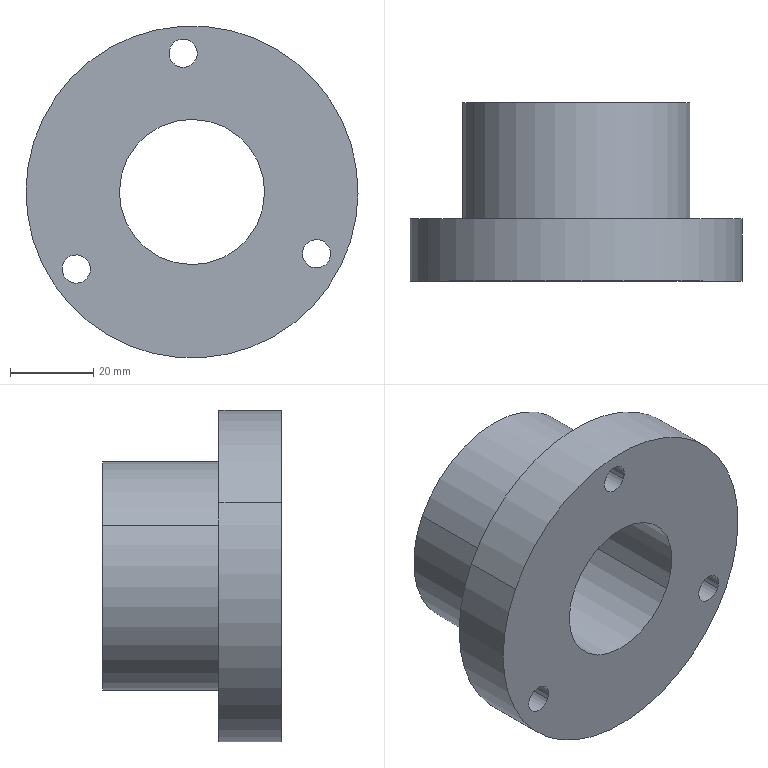Component | SolidWorks | BearingHousing2-1 | 1 solid | 18 faces | box 80 x 43 x 80 mm | volume 88097 mm3 | cylinder 14 | plane 4 | commonest cylinder face diameters 6.8 x6 80 x2 35 x2 47 x2 55 x2
STEP:
#1=COLOUR_RGB('',0.7922,0.8196,0.9333);
#2=FILL_AREA_STYLE_COLOUR('',#1);
#3=FILL_AREA_STYLE('',(#2));
#4=SURFACE_STYLE_FILL_AREA(#3);
#5=SURFACE_SIDE_STYLE('',(#4));
#6=SURFACE_STYLE_USAGE(.BOTH.,#5);
#7=PRESENTATION_STYLE_ASSIGNMENT((#6));
#8=CARTESIAN_POINT('',(-7.394,18.149,5.891));
#9=VERTEX_POINT('',#8);
#10=CARTESIAN_POINT('',(-7.154,18.149,5.772));
#11=VERTEX_POINT('',#10);
#12=CARTESIAN_POINT('',(-7.274,18.149,5.832));
#13=DIRECTION('',(0.,1.,0.));
#14=DIRECTION('',(0.896,0.,-0.4441));
#15=AXIS2_PLACEMENT_3D('',#12,#13,#14);
#16=CIRCLE('',#15,0.1339);
#17=EDGE_CURVE('',#9,#11,#16,.T.);
#18=ORIENTED_EDGE('',*,*,#17,.T.);
#19=CARTESIAN_POINT('',(-7.154,17.558,5.772));
#20=VERTEX_POINT('',#19);
#21=CARTESIAN_POINT('',(-7.154,17.558,5.772));
#22=DIRECTION('',(0.,-1.,0.));
#23=VECTOR('',#22,39.37);
#24=LINE('',#21,#23);
#25=EDGE_CURVE('',#11,#20,#24,.T.);
#26=ORIENTED_EDGE('',*,*,#25,.T.);
#27=CARTESIAN_POINT('',(-7.394,17.558,5.891));
#28=VERTEX_POINT('',#27);
#29=CARTESIAN_POINT('',(-7.274,17.558,5.832));
#30=DIRECTION('',(0.,-1.,0.));
#31=DIRECTION('',(-0.896,0.,0.4441));
#32=AXIS2_PLACEMENT_3D('',#29,#30,#31);
#33=CIRCLE('',#32,0.1339);
#34=EDGE_CURVE('',#20,#28,#33,.T.);
#35=ORIENTED_EDGE('',*,*,#34,.T.);
#36=CARTESIAN_POINT('',(-7.394,17.558,5.891));
#37=DIRECTION('',(0.,-1.,0.));
#38=VECTOR('',#37,39.37);
#39=LINE('',#36,#38);
#40=EDGE_CURVE('',#9,#28,#39,.T.);
#41=ORIENTED_EDGE('',*,*,#40,.F.);
#42=EDGE_LOOP('',(#18,#26,#35,#41));
#43=FACE_OUTER_BOUND('',#42,.T.);
#44=CARTESIAN_POINT('',(-7.274,17.558,5.832));
#45=DIRECTION('',(0.,-1.,0.));
#46=DIRECTION('',(-0.896,0.,0.4441));
#47=AXIS2_PLACEMENT_3D('',#44,#45,#46);
#48=CYLINDRICAL_SURFACE('',#47,0.1339);
#49=ADVANCED_FACE('',(#43),#48,.F.);
#50=CARTESIAN_POINT('',(-8.66,18.149,7.793));
#51=VERTEX_POINT('',#50);
#52=CARTESIAN_POINT('',(-8.42,18.149,7.674));
#53=VERTEX_POINT('',#52);
#54=CARTESIAN_POINT('',(-8.54,18.149,7.734));
#55=DIRECTION('',(0.,1.,0.));
#56=DIRECTION('',(0.896,0.,-0.4441));
#57=AXIS2_PLACEMENT_3D('',#54,#55,#56);
#58=CIRCLE('',#57,0.1339);
#59=EDGE_CURVE('',#51,#53,#58,.T.);
#60=ORIENTED_EDGE('',*,*,#59,.T.);
#61=CARTESIAN_POINT('',(-8.42,17.558,7.674));
#62=VERTEX_POINT('',#61);
#63=CARTESIAN_POINT('',(-8.42,17.558,7.674));
#64=DIRECTION('',(0.,-1.,0.));
#65=VECTOR('',#64,39.37);
#66=LINE('',#63,#65);
#67=EDGE_CURVE('',#53,#62,#66,.T.);
#68=ORIENTED_EDGE('',*,*,#67,.T.);
#69=CARTESIAN_POINT('',(-8.66,17.558,7.793));
#70=VERTEX_POINT('',#69);
#71=CARTESIAN_POINT('',(-8.54,17.558,7.734));
#72=DIRECTION('',(0.,-1.,0.));
#73=DIRECTION('',(-0.896,0.,0.4441));
#74=AXIS2_PLACEMENT_3D('',#71,#72,#73);
#75=CIRCLE('',#74,0.1339);
#76=EDGE_CURVE('',#62,#70,#75,.T.);
#77=ORIENTED_EDGE('',*,*,#76,.T.);
#78=CARTESIAN_POINT('',(-8.66,17.558,7.793));
#79=DIRECTION('',(0.,-1.,0.));
#80=VECTOR('',#79,39.37);
#81=LINE('',#78,#80);
#82=EDGE_CURVE('',#51,#70,#81,.T.);
#83=ORIENTED_EDGE('',*,*,#82,.F.);
#84=EDGE_LOOP('',(#60,#68,#77,#83));
#85=FACE_OUTER_BOUND('',#84,.T.);
#86=CARTESIAN_POINT('',(-8.54,17.558,7.734));
#87=DIRECTION('',(0.,-1.,0.));
#88=DIRECTION('',(-0.896,0.,0.4441));
#89=AXIS2_PLACEMENT_3D('',#86,#87,#88);
#90=CYLINDRICAL_SURFACE('',#89,0.1339);
#91=ADVANCED_FACE('',(#85),#90,.F.);
#92=CARTESIAN_POINT('',(-9.674,18.149,5.746));
#93=VERTEX_POINT('',#92);
#94=CARTESIAN_POINT('',(-9.434,18.149,5.627));
#95=VERTEX_POINT('',#94);
#96=CARTESIAN_POINT('',(-9.554,18.149,5.687));
#97=DIRECTION('',(0.,1.,0.));
#98=DIRECTION('',(0.896,0.,-0.4441));
#99=AXIS2_PLACEMENT_3D('',#96,#97,#98);
#100=CIRCLE('',#99,0.1339);
#101=EDGE_CURVE('',#93,#95,#100,.T.);
#102=ORIENTED_EDGE('',*,*,#101,.T.);
#103=CARTESIAN_POINT('',(-9.434,17.558,5.627));
#104=VERTEX_POINT('',#103);
#105=CARTESIAN_POINT('',(-9.434,17.558,5.627));
#106=DIRECTION('',(0.,-1.,0.));
#107=VECTOR('',#106,39.37);
#108=LINE('',#105,#107);
#109=EDGE_CURVE('',#95,#104,#108,.T.);
#110=ORIENTED_EDGE('',*,*,#109,.T.);
#111=CARTESIAN_POINT('',(-9.674,17.558,5.746));
#112=VERTEX_POINT('',#111);
#113=CARTESIAN_POINT('',(-9.554,17.558,5.687));
#114=DIRECTION('',(0.,-1.,0.));
#115=DIRECTION('',(-0.896,0.,0.4441));
#116=AXIS2_PLACEMENT_3D('',#113,#114,#115);
#117=CIRCLE('',#116,0.1339);
#118=EDGE_CURVE('',#104,#112,#117,.T.);
#119=ORIENTED_EDGE('',*,*,#118,.T.);
#120=CARTESIAN_POINT('',(-9.674,17.558,5.746));
#121=DIRECTION('',(0.,-1.,0.));
#122=VECTOR('',#121,39.37);
#123=LINE('',#120,#122);
#124=EDGE_CURVE('',#93,#112,#123,.T.);
#125=ORIENTED_EDGE('',*,*,#124,.F.);
#126=EDGE_LOOP('',(#102,#110,#119,#125));
#127=FACE_OUTER_BOUND('',#126,.T.);
#128=CARTESIAN_POINT('',(-9.554,17.558,5.687));
#129=DIRECTION('',(0.,-1.,0.));
#130=DIRECTION('',(-0.896,0.,0.4441));
#131=AXIS2_PLACEMENT_3D('',#128,#129,#130);
#132=CYLINDRICAL_SURFACE('',#131,0.1339);
#133=ADVANCED_FACE('',(#127),#132,.F.);
#134=CARTESIAN_POINT('',(-9.867,18.149,7.117));
#135=VERTEX_POINT('',#134);
#136=CARTESIAN_POINT('',(-7.045,18.149,5.718));
#137=VERTEX_POINT('',#136);
#138=CARTESIAN_POINT('',(-8.456,18.149,6.417));
#139=DIRECTION('',(0.,-1.,0.));
#140=DIRECTION('',(-0.896,0.,0.4441));
#141=AXIS2_PLACEMENT_3D('',#138,#139,#140);
#142=CIRCLE('',#141,1.575);
#143=EDGE_CURVE('',#135,#137,#142,.T.);
#144=ORIENTED_EDGE('',*,*,#143,.T.);
#145=CARTESIAN_POINT('',(-7.045,17.558,5.718));
#146=VERTEX_POINT('',#145);
#147=CARTESIAN_POINT('',(-7.045,17.335,5.718));
#148=DIRECTION('',(0.,-1.,0.));
#149=VECTOR('',#148,39.37);
#150=LINE('',#147,#149);
#151=EDGE_CURVE('',#137,#146,#150,.T.);
#152=ORIENTED_EDGE('',*,*,#151,.T.);
#153=CARTESIAN_POINT('',(-9.867,17.558,7.117));
#154=VERTEX_POINT('',#153);
#155=CARTESIAN_POINT('',(-8.456,17.558,6.417));
#156=DIRECTION('',(0.,-1.,0.));
#157=DIRECTION('',(-0.896,0.,0.4441));
#158=AXIS2_PLACEMENT_3D('',#155,#156,#157);
#159=CIRCLE('',#158,1.575);
#160=EDGE_CURVE('',#154,#146,#159,.T.);
#161=ORIENTED_EDGE('',*,*,#160,.F.);
#162=CARTESIAN_POINT('',(-9.867,17.335,7.117));
#163=DIRECTION('',(0.,-1.,0.));
#164=VECTOR('',#163,39.37);
#165=LINE('',#162,#164);
#166=EDGE_CURVE('',#135,#154,#165,.T.);
#167=ORIENTED_EDGE('',*,*,#166,.F.);
#168=EDGE_LOOP('',(#144,#152,#161,#167));
#169=FACE_OUTER_BOUND('',#168,.T.);
#170=CARTESIAN_POINT('',(-8.456,17.335,6.417));
#171=DIRECTION('',(0.,-1.,0.));
#172=DIRECTION('',(-0.896,0.,0.4441));
#173=AXIS2_PLACEMENT_3D('',#170,#171,#172);
#174=CYLINDRICAL_SURFACE('',#173,1.575);
#175=ADVANCED_FACE('',(#169),#174,.T.);
#176=CARTESIAN_POINT('',(-7.839,18.7,6.111));
#177=VERTEX_POINT('',#176);
#178=CARTESIAN_POINT('',(-9.073,18.7,6.723));
#179=VERTEX_POINT('',#178);
#180=CARTESIAN_POINT('',(-8.456,18.7,6.417));
#181=DIRECTION('',(0.,-1.,0.));
#182=DIRECTION('',(-0.896,0.,0.4441));
#183=AXIS2_PLACEMENT_3D('',#180,#181,#182);
#184=CIRCLE('',#183,0.689);
#185=EDGE_CURVE('',#177,#179,#184,.T.);
#186=ORIENTED_EDGE('',*,*,#185,.F.);
#187=CARTESIAN_POINT('',(-7.839,17.558,6.111));
#188=VERTEX_POINT('',#187);
#189=CARTESIAN_POINT('',(-7.839,17.335,6.111));
#190=DIRECTION('',(0.,-1.,0.));
#191=VECTOR('',#190,39.37);
#192=LINE('',#189,#191);
#193=EDGE_CURVE('',#177,#188,#192,.T.);
#194=ORIENTED_EDGE('',*,*,#193,.T.);
#195=CARTESIAN_POINT('',(-9.073,17.558,6.723));
#196=VERTEX_POINT('',#195);
#197=CARTESIAN_POINT('',(-8.456,17.558,6.417));
#198=DIRECTION('',(0.,-1.,0.));
#199=DIRECTION('',(-0.896,0.,0.4441));
#200=AXIS2_PLACEMENT_3D('',#197,#198,#199);
#201=CIRCLE('',#200,0.689);
#202=EDGE_CURVE('',#188,#196,#201,.T.);
#203=ORIENTED_EDGE('',*,*,#202,.T.);
#204=CARTESIAN_POINT('',(-9.073,17.335,6.723));
#205=DIRECTION('',(0.,-1.,0.));
#206=VECTOR('',#205,39.37);
#207=LINE('',#204,#206);
#208=EDGE_CURVE('',#179,#196,#207,.T.);
#209=ORIENTED_EDGE('',*,*,#208,.F.);
#210=EDGE_LOOP('',(#186,#194,#203,#209));
#211=FACE_OUTER_BOUND('',#210,.T.);
#212=CARTESIAN_POINT('',(-8.456,17.335,6.417));
#213=DIRECTION('',(0.,-1.,0.));
#214=DIRECTION('',(-0.896,0.,0.4441));
#215=AXIS2_PLACEMENT_3D('',#212,#213,#214);
#216=CYLINDRICAL_SURFACE('',#215,0.689);
#217=ADVANCED_FACE('',(#211),#216,.F.);
#218=CARTESIAN_POINT('',(-7.627,19.251,6.006));
#219=VERTEX_POINT('',#218);
#220=CARTESIAN_POINT('',(-9.285,19.251,6.828));
#221=VERTEX_POINT('',#220);
#222=CARTESIAN_POINT('',(-8.456,19.251,6.417));
#223=DIRECTION('',(0.,-1.,0.));
#224=DIRECTION('',(-0.896,0.,0.4441));
#225=AXIS2_PLACEMENT_3D('',#222,#223,#224);
#226=CIRCLE('',#225,0.9252);
#227=EDGE_CURVE('',#219,#221,#226,.T.);
#228=ORIENTED_EDGE('',*,*,#227,.F.);
#229=CARTESIAN_POINT('',(-7.627,18.7,6.006));
#230=VERTEX_POINT('',#229);
#231=CARTESIAN_POINT('',(-7.627,17.335,6.006));
#232=DIRECTION('',(0.,-1.,0.));
#233=VECTOR('',#232,39.37);
#234=LINE('',#231,#233);
#235=EDGE_CURVE('',#219,#230,#234,.T.);
#236=ORIENTED_EDGE('',*,*,#235,.T.);
#237=CARTESIAN_POINT('',(-9.285,18.7,6.828));
#238=VERTEX_POINT('',#237);
#239=CARTESIAN_POINT('',(-8.456,18.7,6.417));
#240=DIRECTION('',(0.,-1.,0.));
#241=DIRECTION('',(-0.896,0.,0.4441));
#242=AXIS2_PLACEMENT_3D('',#239,#240,#241);
#243=CIRCLE('',#242,0.9252);
#244=EDGE_CURVE('',#230,#238,#243,.T.);
#245=ORIENTED_EDGE('',*,*,#244,.T.);
#246=CARTESIAN_POINT('',(-9.285,17.335,6.828));
#247=DIRECTION('',(0.,-1.,0.));
#248=VECTOR('',#247,39.37);
#249=LINE('',#246,#248);
#250=EDGE_CURVE('',#221,#238,#249,.T.);
#251=ORIENTED_EDGE('',*,*,#250,.F.);
#252=EDGE_LOOP('',(#228,#236,#245,#251));
#253=FACE_OUTER_BOUND('',#252,.T.);
#254=CARTESIAN_POINT('',(-8.456,17.335,6.417));
#255=DIRECTION('',(0.,-1.,0.));
#256=DIRECTION('',(-0.896,0.,0.4441));
#257=AXIS2_PLACEMENT_3D('',#254,#255,#256);
#258=CYLINDRICAL_SURFACE('',#257,0.9252);
#259=ADVANCED_FACE('',(#253),#258,.F.);
#260=CARTESIAN_POINT('',(-9.426,19.251,6.898));
#261=VERTEX_POINT('',#260);
#262=CARTESIAN_POINT('',(-7.486,19.251,5.937));
#263=VERTEX_POINT('',#262);
#264=CARTESIAN_POINT('',(-8.456,19.251,6.417));
#265=DIRECTION('',(0.,-1.,0.));
#266=DIRECTION('',(-0.896,0.,0.4441));
#267=AXIS2_PLACEMENT_3D('',#264,#265,#266);
#268=CIRCLE('',#267,1.083);
#269=EDGE_CURVE('',#261,#263,#268,.T.);
#270=ORIENTED_EDGE('',*,*,#269,.T.);
#271=CARTESIAN_POINT('',(-7.486,18.149,5.937));
#272=VERTEX_POINT('',#271);
#273=CARTESIAN_POINT('',(-7.486,17.335,5.937));
#274=DIRECTION('',(0.,-1.,0.));
#275=VECTOR('',#274,39.37);
#276=LINE('',#273,#275);
#277=EDGE_CURVE('',#263,#272,#276,.T.);
#278=ORIENTED_EDGE('',*,*,#277,.T.);
#279=CARTESIAN_POINT('',(-9.426,18.149,6.898));
#280=VERTEX_POINT('',#279);
#281=CARTESIAN_POINT('',(-8.456,18.149,6.417));
#282=DIRECTION('',(0.,-1.,0.));
#283=DIRECTION('',(-0.896,0.,0.4441));
#284=AXIS2_PLACEMENT_3D('',#281,#282,#283);
#285=CIRCLE('',#284,1.083);
#286=EDGE_CURVE('',#280,#272,#285,.T.);
#287=ORIENTED_EDGE('',*,*,#286,.F.);
#288=CARTESIAN_POINT('',(-9.426,17.335,6.898));
#289=DIRECTION('',(0.,-1.,0.));
#290=VECTOR('',#289,39.37);
#291=LINE('',#288,#290);
#292=EDGE_CURVE('',#261,#280,#291,.T.);
#293=ORIENTED_EDGE('',*,*,#292,.F.);
#294=EDGE_LOOP('',(#270,#278,#287,#293));
#295=FACE_OUTER_BOUND('',#294,.T.);
#296=CARTESIAN_POINT('',(-8.456,17.335,6.417));
#297=DIRECTION('',(0.,-1.,0.));
#298=DIRECTION('',(-0.896,0.,0.4441));
#299=AXIS2_PLACEMENT_3D('',#296,#297,#298);
#300=CYLINDRICAL_SURFACE('',#299,1.083);
#301=ADVANCED_FACE('',(#295),#300,.T.);
#302=ORIENTED_EDGE('',*,*,#277,.F.);
#303=CARTESIAN_POINT('',(-8.456,19.251,6.417));
#304=DIRECTION('',(0.,-1.,0.));
#305=DIRECTION('',(-0.896,0.,0.4441));
#306=AXIS2_PLACEMENT_3D('',#303,#304,#305);
#307=CIRCLE('',#306,1.083);
#308=EDGE_CURVE('',#263,#261,#307,.T.);
#309=ORIENTED_EDGE('',*,*,#308,.T.);
#310=ORIENTED_EDGE('',*,*,#292,.T.);
#311=CARTESIAN_POINT('',(-8.456,18.149,6.417));
#312=DIRECTION('',(0.,-1.,0.));
#313=DIRECTION('',(-0.896,0.,0.4441));
#314=AXIS2_PLACEMENT_3D('',#311,#312,#313);
#315=CIRCLE('',#314,1.083);
#316=EDGE_CURVE('',#272,#280,#315,.T.);
#317=ORIENTED_EDGE('',*,*,#316,.F.);
#318=EDGE_LOOP('',(#302,#309,#310,#317));
#319=FACE_OUTER_BOUND('',#318,.T.);
#320=CARTESIAN_POINT('',(-8.456,17.335,6.417));
#321=DIRECTION('',(0.,-1.,0.));
#322=DIRECTION('',(-0.896,0.,0.4441));
#323=AXIS2_PLACEMENT_3D('',#320,#321,#322);
#324=CYLINDRICAL_SURFACE('',#323,1.083);
#325=ADVANCED_FACE('',(#319),#324,.T.);
#326=CARTESIAN_POINT('',(-8.456,19.251,6.417));
#327=DIRECTION('',(0.,-1.,0.));
#328=DIRECTION('',(-0.896,0.,0.4441));
#329=AXIS2_PLACEMENT_3D('',#326,#327,#328);
#330=CIRCLE('',#329,0.9252);
#331=EDGE_CURVE('',#221,#219,#330,.T.);
#332=ORIENTED_EDGE('',*,*,#331,.T.);
#333=ORIENTED_EDGE('',*,*,#227,.T.);
#334=EDGE_LOOP('',(#332,#333));
#335=FACE_BOUND('',#334,.T.);
#336=ORIENTED_EDGE('',*,*,#269,.F.);
#337=ORIENTED_EDGE('',*,*,#308,.F.);
#338=EDGE_LOOP('',(#336,#337));
#339=FACE_OUTER_BOUND('',#338,.T.);
#340=CARTESIAN_POINT('',(-9.285,19.251,6.828));
#341=DIRECTION('',(0.,1.,0.));
#342=DIRECTION('',(0.896,0.,-0.4441));
#343=AXIS2_PLACEMENT_3D('',#340,#341,#342);
#344=PLANE('',#343);
#345=ADVANCED_FACE('',(#335,#339),#344,.T.);
#346=ORIENTED_EDGE('',*,*,#235,.F.);
#347=ORIENTED_EDGE('',*,*,#331,.F.);
#348=ORIENTED_EDGE('',*,*,#250,.T.);
#349=CARTESIAN_POINT('',(-8.456,18.7,6.417));
#350=DIRECTION('',(0.,-1.,0.));
#351=DIRECTION('',(-0.896,0.,0.4441));
#352=AXIS2_PLACEMENT_3D('',#349,#350,#351);
#353=CIRCLE('',#352,0.9252);
#354=EDGE_CURVE('',#238,#230,#353,.T.);
#355=ORIENTED_EDGE('',*,*,#354,.T.);
#356=EDGE_LOOP('',(#346,#347,#348,#355));
#357=FACE_OUTER_BOUND('',#356,.T.);
#358=CARTESIAN_POINT('',(-8.456,17.335,6.417));
#359=DIRECTION('',(0.,-1.,0.));
#360=DIRECTION('',(-0.896,0.,0.4441));
#361=AXIS2_PLACEMENT_3D('',#358,#359,#360);
#362=CYLINDRICAL_SURFACE('',#361,0.9252);
#363=ADVANCED_FACE('',(#357),#362,.F.);
#364=CARTESIAN_POINT('',(-8.456,18.7,6.417));
#365=DIRECTION('',(0.,-1.,0.));
#366=DIRECTION('',(-0.896,0.,0.4441));
#367=AXIS2_PLACEMENT_3D('',#364,#365,#366);
#368=CIRCLE('',#367,0.689);
#369=EDGE_CURVE('',#179,#177,#368,.T.);
#370=ORIENTED_EDGE('',*,*,#369,.T.);
#371=ORIENTED_EDGE('',*,*,#185,.T.);
#372=EDGE_LOOP('',(#370,#371));
#373=FACE_BOUND('',#372,.T.);
#374=ORIENTED_EDGE('',*,*,#354,.F.);
#375=ORIENTED_EDGE('',*,*,#244,.F.);
#376=EDGE_LOOP('',(#374,#375));
#377=FACE_OUTER_BOUND('',#376,.T.);
#378=CARTESIAN_POINT('',(-9.285,18.7,6.828));
#379=DIRECTION('',(0.,1.,0.));
#380=DIRECTION('',(0.896,0.,-0.4441));
#381=AXIS2_PLACEMENT_3D('',#378,#379,#380);
#382=PLANE('',#381);
#383=ADVANCED_FACE('',(#373,#377),#382,.T.);
#384=ORIENTED_EDGE('',*,*,#193,.F.);
#385=ORIENTED_EDGE('',*,*,#369,.F.);
#386=ORIENTED_EDGE('',*,*,#208,.T.);
#387=CARTESIAN_POINT('',(-8.456,17.558,6.417));
#388=DIRECTION('',(0.,-1.,0.));
#389=DIRECTION('',(-0.896,0.,0.4441));
#390=AXIS2_PLACEMENT_3D('',#387,#388,#389);
#391=CIRCLE('',#390,0.689);
#392=EDGE_CURVE('',#196,#188,#391,.T.);
#393=ORIENTED_EDGE('',*,*,#392,.T.);
#394=EDGE_LOOP('',(#384,#385,#386,#393));
#395=FACE_OUTER_BOUND('',#394,.T.);
#396=CARTESIAN_POINT('',(-8.456,17.335,6.417));
#397=DIRECTION('',(0.,-1.,0.));
#398=DIRECTION('',(-0.896,0.,0.4441));
#399=AXIS2_PLACEMENT_3D('',#396,#397,#398);
#400=CYLINDRICAL_SURFACE('',#399,0.689);
#401=ADVANCED_FACE('',(#395),#400,.F.);
#402=CARTESIAN_POINT('',(-7.274,17.558,5.832));
#403=DIRECTION('',(0.,-1.,0.));
#404=DIRECTION('',(-0.896,0.,0.4441));
#405=AXIS2_PLACEMENT_3D('',#402,#403,#404);
#406=CIRCLE('',#405,0.1339);
#407=EDGE_CURVE('',#28,#20,#406,.T.);
#408=ORIENTED_EDGE('',*,*,#407,.F.);
#409=ORIENTED_EDGE('',*,*,#34,.F.);
#410=EDGE_LOOP('',(#408,#409));
#411=FACE_BOUND('',#410,.T.);
#412=CARTESIAN_POINT('',(-8.54,17.558,7.734));
#413=DIRECTION('',(0.,-1.,0.));
#414=DIRECTION('',(-0.896,0.,0.4441));
#415=AXIS2_PLACEMENT_3D('',#412,#413,#414);
#416=CIRCLE('',#415,0.1339);
#417=EDGE_CURVE('',#70,#62,#416,.T.);
#418=ORIENTED_EDGE('',*,*,#417,.F.);
#419=ORIENTED_EDGE('',*,*,#76,.F.);
#420=EDGE_LOOP('',(#418,#419));
#421=FACE_BOUND('',#420,.T.);
#422=CARTESIAN_POINT('',(-9.554,17.558,5.687));
#423=DIRECTION('',(0.,-1.,0.));
#424=DIRECTION('',(-0.896,0.,0.4441));
#425=AXIS2_PLACEMENT_3D('',#422,#423,#424);
#426=CIRCLE('',#425,0.1339);
#427=EDGE_CURVE('',#112,#104,#426,.T.);
#428=ORIENTED_EDGE('',*,*,#427,.F.);
#429=ORIENTED_EDGE('',*,*,#118,.F.);
#430=EDGE_LOOP('',(#428,#429));
#431=FACE_BOUND('',#430,.T.);
#432=ORIENTED_EDGE('',*,*,#160,.T.);
#433=CARTESIAN_POINT('',(-8.456,17.558,6.417));
#434=DIRECTION('',(0.,-1.,0.));
#435=DIRECTION('',(-0.896,0.,0.4441));
#436=AXIS2_PLACEMENT_3D('',#433,#434,#435);
#437=CIRCLE('',#436,1.575);
#438=EDGE_CURVE('',#146,#154,#437,.T.);
#439=ORIENTED_EDGE('',*,*,#438,.T.);
#440=EDGE_LOOP('',(#432,#439));
#441=FACE_OUTER_BOUND('',#440,.T.);
#442=ORIENTED_EDGE('',*,*,#392,.F.);
#443=ORIENTED_EDGE('',*,*,#202,.F.);
#444=EDGE_LOOP('',(#442,#443));
#445=FACE_BOUND('',#444,.T.);
#446=CARTESIAN_POINT('',(-9.867,17.558,7.117));
#447=DIRECTION('',(0.,-1.,0.));
#448=DIRECTION('',(-0.896,0.,0.4441));
#449=AXIS2_PLACEMENT_3D('',#446,#447,#448);
#450=PLANE('',#449);
#451=ADVANCED_FACE('',(#411,#421,#431,#441,#445),#450,.T.);
#452=ORIENTED_EDGE('',*,*,#151,.F.);
#453=CARTESIAN_POINT('',(-8.456,18.149,6.417));
#454=DIRECTION('',(0.,-1.,0.));
#455=DIRECTION('',(-0.896,0.,0.4441));
#456=AXIS2_PLACEMENT_3D('',#453,#454,#455);
#457=CIRCLE('',#456,1.575);
#458=EDGE_CURVE('',#137,#135,#457,.T.);
#459=ORIENTED_EDGE('',*,*,#458,.T.);
#460=ORIENTED_EDGE('',*,*,#166,.T.);
#461=ORIENTED_EDGE('',*,*,#438,.F.);
#462=EDGE_LOOP('',(#452,#459,#460,#461));
#463=FACE_OUTER_BOUND('',#462,.T.);
#464=CARTESIAN_POINT('',(-8.456,17.335,6.417));
#465=DIRECTION('',(0.,-1.,0.));
#466=DIRECTION('',(-0.896,0.,0.4441));
#467=AXIS2_PLACEMENT_3D('',#464,#465,#466);
#468=CYLINDRICAL_SURFACE('',#467,1.575);
#469=ADVANCED_FACE('',(#463),#468,.T.);
#470=ORIENTED_EDGE('',*,*,#17,.F.);
#471=CARTESIAN_POINT('',(-7.274,18.149,5.832));
#472=DIRECTION('',(0.,1.,0.));
#473=DIRECTION('',(0.896,0.,-0.4441));
#474=AXIS2_PLACEMENT_3D('',#471,#472,#473);
#475=CIRCLE('',#474,0.1339);
#476=EDGE_CURVE('',#11,#9,#475,.T.);
#477=ORIENTED_EDGE('',*,*,#476,.F.);
#478=EDGE_LOOP('',(#470,#477));
#479=FACE_BOUND('',#478,.T.);
#480=ORIENTED_EDGE('',*,*,#59,.F.);
#481=CARTESIAN_POINT('',(-8.54,18.149,7.734));
#482=DIRECTION('',(0.,1.,0.));
#483=DIRECTION('',(0.896,0.,-0.4441));
#484=AXIS2_PLACEMENT_3D('',#481,#482,#483);
#485=CIRCLE('',#484,0.1339);
#486=EDGE_CURVE('',#53,#51,#485,.T.);
#487=ORIENTED_EDGE('',*,*,#486,.F.);
#488=EDGE_LOOP('',(#480,#487));
#489=FACE_BOUND('',#488,.T.);
#490=ORIENTED_EDGE('',*,*,#101,.F.);
#491=CARTESIAN_POINT('',(-9.554,18.149,5.687));
#492=DIRECTION('',(0.,1.,0.));
#493=DIRECTION('',(0.896,0.,-0.4441));
#494=AXIS2_PLACEMENT_3D('',#491,#492,#493);
#495=CIRCLE('',#494,0.1339);
#496=EDGE_CURVE('',#95,#93,#495,.T.);
#497=ORIENTED_EDGE('',*,*,#496,.F.);
#498=EDGE_LOOP('',(#490,#497));
#499=FACE_BOUND('',#498,.T.);
#500=ORIENTED_EDGE('',*,*,#286,.T.);
#501=ORIENTED_EDGE('',*,*,#316,.T.);
#502=EDGE_LOOP('',(#500,#501));
#503=FACE_BOUND('',#502,.T.);
#504=ORIENTED_EDGE('',*,*,#143,.F.);
#505=ORIENTED_EDGE('',*,*,#458,.F.);
#506=EDGE_LOOP('',(#504,#505));
#507=FACE_OUTER_BOUND('',#506,.T.);
#508=CARTESIAN_POINT('',(-9.426,18.149,6.898));
#509=DIRECTION('',(0.,1.,0.));
#510=DIRECTION('',(0.896,0.,-0.4441));
#511=AXIS2_PLACEMENT_3D('',#508,#509,#510);
#512=PLANE('',#511);
#513=ADVANCED_FACE('',(#479,#489,#499,#503,#507),#512,.T.);
#514=ORIENTED_EDGE('',*,*,#109,.F.);
#515=ORIENTED_EDGE('',*,*,#496,.T.);
#516=ORIENTED_EDGE('',*,*,#124,.T.);
#517=ORIENTED_EDGE('',*,*,#427,.T.);
#518=EDGE_LOOP('',(#514,#515,#516,#517));
#519=FACE_OUTER_BOUND('',#518,.T.);
#520=CARTESIAN_POINT('',(-9.554,17.558,5.687));
#521=DIRECTION('',(0.,-1.,0.));
#522=DIRECTION('',(-0.896,0.,0.4441));
#523=AXIS2_PLACEMENT_3D('',#520,#521,#522);
#524=CYLINDRICAL_SURFACE('',#523,0.1339);
#525=ADVANCED_FACE('',(#519),#524,.F.);
#526=ORIENTED_EDGE('',*,*,#67,.F.);
#527=ORIENTED_EDGE('',*,*,#486,.T.);
#528=ORIENTED_EDGE('',*,*,#82,.T.);
#529=ORIENTED_EDGE('',*,*,#417,.T.);
#530=EDGE_LOOP('',(#526,#527,#528,#529));
#531=FACE_OUTER_BOUND('',#530,.T.);
#532=CARTESIAN_POINT('',(-8.54,17.558,7.734));
#533=DIRECTION('',(0.,-1.,0.));
#534=DIRECTION('',(-0.896,0.,0.4441));
#535=AXIS2_PLACEMENT_3D('',#532,#533,#534);
#536=CYLINDRICAL_SURFACE('',#535,0.1339);
#537=ADVANCED_FACE('',(#531),#536,.F.);
#538=ORIENTED_EDGE('',*,*,#25,.F.);
#539=ORIENTED_EDGE('',*,*,#476,.T.);
#540=ORIENTED_EDGE('',*,*,#40,.T.);
#541=ORIENTED_EDGE('',*,*,#407,.T.);
#542=EDGE_LOOP('',(#538,#539,#540,#541));
#543=FACE_OUTER_BOUND('',#542,.T.);
#544=CARTESIAN_POINT('',(-7.274,17.558,5.832));
#545=DIRECTION('',(0.,-1.,0.));
#546=DIRECTION('',(-0.896,0.,0.4441));
#547=AXIS2_PLACEMENT_3D('',#544,#545,#546);
#548=CYLINDRICAL_SURFACE('',#547,0.1339);
#549=ADVANCED_FACE('',(#543),#548,.F.);
#550=CLOSED_SHELL('',(#49,#91,#133,#175,#217,#259,#301,#325,#345,#363,#383,#401,#451,#469,#513,#525,#537,#549));
#551=MANIFOLD_SOLID_BREP('',#550);
#552=STYLED_ITEM('',(#7),#551);
#553=(LENGTH_UNIT()NAMED_UNIT(*)SI_UNIT($,.METRE.));
#554=LENGTH_MEASURE_WITH_UNIT(LENGTH_MEASURE(0.0254),#553);
#555=DIMENSIONAL_EXPONENTS(1.,0.,0.,0.,0.,0.,0.);
#556=(CONVERSION_BASED_UNIT('',#554)LENGTH_UNIT()NAMED_UNIT(#555));
#557=UNCERTAINTY_MEASURE_WITH_UNIT(LENGTH_MEASURE(0.00001),#556,'','');
#558=(NAMED_UNIT(*)PLANE_ANGLE_UNIT()SI_UNIT($,.RADIAN.));
#559=(NAMED_UNIT(*)SI_UNIT($,.STERADIAN.)SOLID_ANGLE_UNIT());
#560=(GEOMETRIC_REPRESENTATION_CONTEXT(3)GLOBAL_UNCERTAINTY_ASSIGNED_CONTEXT((#557))GLOBAL_UNIT_ASSIGNED_CONTEXT((#556,#558,#559))REPRESENTATION_CONTEXT('',''));
#561=MECHANICAL_DESIGN_GEOMETRIC_PRESENTATION_REPRESENTATION('',(#552),#560);
#562=CARTESIAN_POINT('',(0.,0.,0.));
#563=DIRECTION('',(0.,0.,1.));
#564=DIRECTION('',(1.,0.,0.));
#565=AXIS2_PLACEMENT_3D('',#562,#563,#564);
#566=(LENGTH_UNIT()NAMED_UNIT(*)SI_UNIT($,.METRE.));
#567=LENGTH_MEASURE_WITH_UNIT(LENGTH_MEASURE(0.0254),#566);
#568=DIMENSIONAL_EXPONENTS(1.,0.,0.,0.,0.,0.,0.);
#569=(CONVERSION_BASED_UNIT('',#567)LENGTH_UNIT()NAMED_UNIT(#568));
#570=UNCERTAINTY_MEASURE_WITH_UNIT(LENGTH_MEASURE(0.00001),#569,'','');
#571=(NAMED_UNIT(*)PLANE_ANGLE_UNIT()SI_UNIT($,.RADIAN.));
#572=(NAMED_UNIT(*)SI_UNIT($,.STERADIAN.)SOLID_ANGLE_UNIT());
#573=(GEOMETRIC_REPRESENTATION_CONTEXT(3)GLOBAL_UNCERTAINTY_ASSIGNED_CONTEXT((#570))GLOBAL_UNIT_ASSIGNED_CONTEXT((#569,#571,#572))REPRESENTATION_CONTEXT('',''));
#574=ADVANCED_BREP_SHAPE_REPRESENTATION('',(#551,#565),#573);
#575=PRESENTATION_LAYER_ASSIGNMENT('','',(#552));